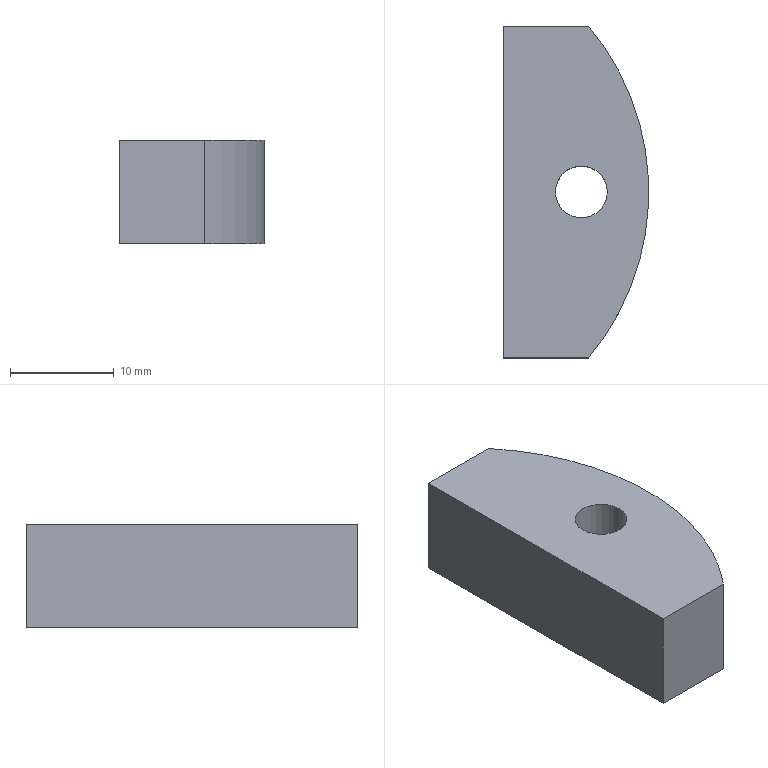Component | NX | CURVED_CLAMP_BLOCK | 1 solid | 7 faces | box 14 x 32 x 10 mm | volume 3698 mm3 | plane 5 | cylinder 2 | commonest cylinder face diameters 50 x1 5 x1
STEP:
#1=CARTESIAN_POINT('',(0.,0.,0.));
#2=DIRECTION('',(0.,0.,1.));
#3=DIRECTION('',(1.,0.,0.));
#4=AXIS2_PLACEMENT_3D('',#1,#2,#3);
#5=CARTESIAN_POINT('',(33.,15.25,-21.5));
#6=VERTEX_POINT('',#5);
#7=CARTESIAN_POINT('',(33.,-16.75,-21.5));
#8=VERTEX_POINT('',#7);
#9=CARTESIAN_POINT('',(33.,15.25,-21.5));
#10=DIRECTION('',(0.,-1.,0.));
#11=VECTOR('',#10,1.);
#12=LINE('',#9,#11);
#13=CARTESIAN_POINT('',(33.,15.25,-11.5));
#14=DIRECTION('',(1.,0.,0.));
#15=DIRECTION('',(-0.,1.,0.));
#16=AXIS2_PLACEMENT_3D('',#13,#14,#15);
#17=PLANE('',#16);
#18=CARTESIAN_POINT('',(0.,-10.));
#19=DIRECTION('',(-1.,0.));
#20=VECTOR('',#19,1.);
#21=LINE('',#18,#20);
#22=(GEOMETRIC_REPRESENTATION_CONTEXT(2)PARAMETRIC_REPRESENTATION_CONTEXT()REPRESENTATION_CONTEXT('',''));
#23=DEFINITIONAL_REPRESENTATION('',(#21),#22);
#24=PCURVE('',#17,#23);
#25=CARTESIAN_POINT('',(22.,-0.75,-21.5));
#26=DIRECTION('',(0.,0.,1.));
#27=DIRECTION('',(1.,0.,0.));
#28=AXIS2_PLACEMENT_3D('',#25,#26,#27);
#29=PLANE('',#28);
#30=CARTESIAN_POINT('',(11.,16.));
#31=DIRECTION('',(0.,-1.));
#32=VECTOR('',#31,1.);
#33=LINE('',#30,#32);
#34=(GEOMETRIC_REPRESENTATION_CONTEXT(2)PARAMETRIC_REPRESENTATION_CONTEXT()REPRESENTATION_CONTEXT('',''));
#35=DEFINITIONAL_REPRESENTATION('',(#33),#34);
#36=PCURVE('',#29,#35);
#37=SURFACE_CURVE('',#12,(#24,#36),.PCURVE_S1.);
#38=EDGE_CURVE('',#6,#8,#37,.T.);
#39=ORIENTED_EDGE('',*,*,#38,.T.);
#40=CARTESIAN_POINT('',(33.,-16.75,-11.5));
#41=VERTEX_POINT('',#40);
#42=CARTESIAN_POINT('',(33.,-16.75,-11.5));
#43=DIRECTION('',(0.,0.,-1.));
#44=VECTOR('',#43,1.);
#45=LINE('',#42,#44);
#46=CARTESIAN_POINT('',(-32.,0.));
#47=DIRECTION('',(0.,-1.));
#48=VECTOR('',#47,1.);
#49=LINE('',#46,#48);
#50=(GEOMETRIC_REPRESENTATION_CONTEXT(2)PARAMETRIC_REPRESENTATION_CONTEXT()REPRESENTATION_CONTEXT('',''));
#51=DEFINITIONAL_REPRESENTATION('',(#49),#50);
#52=PCURVE('',#17,#51);
#53=CARTESIAN_POINT('',(33.,-16.75,-11.5));
#54=DIRECTION('',(0.,1.,0.));
#55=DIRECTION('',(0.,0.,1.));
#56=AXIS2_PLACEMENT_3D('',#53,#54,#55);
#57=PLANE('',#56);
#58=CARTESIAN_POINT('',(0.,0.));
#59=DIRECTION('',(-1.,0.));
#60=VECTOR('',#59,1.);
#61=LINE('',#58,#60);
#62=(GEOMETRIC_REPRESENTATION_CONTEXT(2)PARAMETRIC_REPRESENTATION_CONTEXT()REPRESENTATION_CONTEXT('',''));
#63=DEFINITIONAL_REPRESENTATION('',(#61),#62);
#64=PCURVE('',#57,#63);
#65=SURFACE_CURVE('',#45,(#52,#64),.PCURVE_S1.);
#66=EDGE_CURVE('',#41,#8,#65,.T.);
#67=ORIENTED_EDGE('',*,*,#66,.F.);
#68=CARTESIAN_POINT('',(33.,15.25,-11.5));
#69=VERTEX_POINT('',#68);
#70=CARTESIAN_POINT('',(33.,15.25,-11.5));
#71=DIRECTION('',(0.,-1.,0.));
#72=VECTOR('',#71,1.);
#73=LINE('',#70,#72);
#74=CARTESIAN_POINT('',(0.,0.));
#75=DIRECTION('',(-1.,0.));
#76=VECTOR('',#75,1.);
#77=LINE('',#74,#76);
#78=(GEOMETRIC_REPRESENTATION_CONTEXT(2)PARAMETRIC_REPRESENTATION_CONTEXT()REPRESENTATION_CONTEXT('',''));
#79=DEFINITIONAL_REPRESENTATION('',(#77),#78);
#80=PCURVE('',#17,#79);
#81=CARTESIAN_POINT('',(22.,-0.75,-11.5));
#82=DIRECTION('',(0.,0.,1.));
#83=DIRECTION('',(1.,0.,0.));
#84=AXIS2_PLACEMENT_3D('',#81,#82,#83);
#85=PLANE('',#84);
#86=CARTESIAN_POINT('',(11.,16.));
#87=DIRECTION('',(0.,-1.));
#88=VECTOR('',#87,1.);
#89=LINE('',#86,#88);
#90=(GEOMETRIC_REPRESENTATION_CONTEXT(2)PARAMETRIC_REPRESENTATION_CONTEXT()REPRESENTATION_CONTEXT('',''));
#91=DEFINITIONAL_REPRESENTATION('',(#89),#90);
#92=PCURVE('',#85,#91);
#93=SURFACE_CURVE('',#73,(#80,#92),.PCURVE_S1.);
#94=EDGE_CURVE('',#69,#41,#93,.T.);
#95=ORIENTED_EDGE('',*,*,#94,.F.);
#96=CARTESIAN_POINT('',(33.,15.25,-11.5));
#97=DIRECTION('',(0.,0.,-1.));
#98=VECTOR('',#97,1.);
#99=LINE('',#96,#98);
#100=CARTESIAN_POINT('',(0.,0.));
#101=DIRECTION('',(0.,-1.));
#102=VECTOR('',#101,1.);
#103=LINE('',#100,#102);
#104=(GEOMETRIC_REPRESENTATION_CONTEXT(2)PARAMETRIC_REPRESENTATION_CONTEXT()REPRESENTATION_CONTEXT('',''));
#105=DEFINITIONAL_REPRESENTATION('',(#103),#104);
#106=PCURVE('',#17,#105);
#107=CARTESIAN_POINT('',(41.209,15.25,-11.5));
#108=DIRECTION('',(0.,-1.,0.));
#109=DIRECTION('',(0.,0.,-1.));
#110=AXIS2_PLACEMENT_3D('',#107,#108,#109);
#111=PLANE('',#110);
#112=CARTESIAN_POINT('',(0.,-8.209));
#113=DIRECTION('',(1.,0.));
#114=VECTOR('',#113,1.);
#115=LINE('',#112,#114);
#116=(GEOMETRIC_REPRESENTATION_CONTEXT(2)PARAMETRIC_REPRESENTATION_CONTEXT()REPRESENTATION_CONTEXT('',''));
#117=DEFINITIONAL_REPRESENTATION('',(#115),#116);
#118=PCURVE('',#111,#117);
#119=SURFACE_CURVE('',#99,(#106,#118),.PCURVE_S1.);
#120=EDGE_CURVE('',#69,#6,#119,.T.);
#121=ORIENTED_EDGE('',*,*,#120,.T.);
#122=EDGE_LOOP('',(#39,#67,#95,#121));
#123=FACE_BOUND('',#122,.T.);
#124=ADVANCED_FACE('',(#123),#17,.F.);
#125=CARTESIAN_POINT('',(41.209,-16.75,-21.5));
#126=VERTEX_POINT('',#125);
#127=CARTESIAN_POINT('',(33.,-16.75,-21.5));
#128=DIRECTION('',(1.,0.,0.));
#129=VECTOR('',#128,1.);
#130=LINE('',#127,#129);
#131=CARTESIAN_POINT('',(-10.,0.));
#132=DIRECTION('',(0.,1.));
#133=VECTOR('',#132,1.);
#134=LINE('',#131,#133);
#135=(GEOMETRIC_REPRESENTATION_CONTEXT(2)PARAMETRIC_REPRESENTATION_CONTEXT()REPRESENTATION_CONTEXT('',''));
#136=DEFINITIONAL_REPRESENTATION('',(#134),#135);
#137=PCURVE('',#57,#136);
#138=CARTESIAN_POINT('',(11.,-16.));
#139=DIRECTION('',(1.,0.));
#140=VECTOR('',#139,1.);
#141=LINE('',#138,#140);
#142=(GEOMETRIC_REPRESENTATION_CONTEXT(2)PARAMETRIC_REPRESENTATION_CONTEXT()REPRESENTATION_CONTEXT('',''));
#143=DEFINITIONAL_REPRESENTATION('',(#141),#142);
#144=PCURVE('',#29,#143);
#145=SURFACE_CURVE('',#130,(#137,#144),.PCURVE_S1.);
#146=EDGE_CURVE('',#8,#126,#145,.T.);
#147=ORIENTED_EDGE('',*,*,#146,.T.);
#148=CARTESIAN_POINT('',(41.209,-16.75,-11.5));
#149=VERTEX_POINT('',#148);
#150=CARTESIAN_POINT('',(41.209,-16.75,-11.5));
#151=DIRECTION('',(0.,0.,-1.));
#152=VECTOR('',#151,1.);
#153=LINE('',#150,#152);
#154=CARTESIAN_POINT('',(0.,8.209));
#155=DIRECTION('',(-1.,0.));
#156=VECTOR('',#155,1.);
#157=LINE('',#154,#156);
#158=(GEOMETRIC_REPRESENTATION_CONTEXT(2)PARAMETRIC_REPRESENTATION_CONTEXT()REPRESENTATION_CONTEXT('',''));
#159=DEFINITIONAL_REPRESENTATION('',(#157),#158);
#160=PCURVE('',#57,#159);
#161=CARTESIAN_POINT('',(22.,-0.75,-11.5));
#162=DIRECTION('',(0.,0.,-1.));
#163=DIRECTION('',(-1.,0.,0.));
#164=AXIS2_PLACEMENT_3D('',#161,#162,#163);
#165=CYLINDRICAL_SURFACE('',#164,25.);
#166=CARTESIAN_POINT('',(3.836,0.));
#167=DIRECTION('',(0.,1.));
#168=VECTOR('',#167,1.);
#169=LINE('',#166,#168);
#170=(GEOMETRIC_REPRESENTATION_CONTEXT(2)PARAMETRIC_REPRESENTATION_CONTEXT()REPRESENTATION_CONTEXT('',''));
#171=DEFINITIONAL_REPRESENTATION('',(#169),#170);
#172=PCURVE('',#165,#171);
#173=SURFACE_CURVE('',#153,(#160,#172),.PCURVE_S1.);
#174=EDGE_CURVE('',#149,#126,#173,.T.);
#175=ORIENTED_EDGE('',*,*,#174,.F.);
#176=CARTESIAN_POINT('',(33.,-16.75,-11.5));
#177=DIRECTION('',(1.,0.,0.));
#178=VECTOR('',#177,1.);
#179=LINE('',#176,#178);
#180=CARTESIAN_POINT('',(0.,0.));
#181=DIRECTION('',(0.,1.));
#182=VECTOR('',#181,1.);
#183=LINE('',#180,#182);
#184=(GEOMETRIC_REPRESENTATION_CONTEXT(2)PARAMETRIC_REPRESENTATION_CONTEXT()REPRESENTATION_CONTEXT('',''));
#185=DEFINITIONAL_REPRESENTATION('',(#183),#184);
#186=PCURVE('',#57,#185);
#187=CARTESIAN_POINT('',(11.,-16.));
#188=DIRECTION('',(1.,0.));
#189=VECTOR('',#188,1.);
#190=LINE('',#187,#189);
#191=(GEOMETRIC_REPRESENTATION_CONTEXT(2)PARAMETRIC_REPRESENTATION_CONTEXT()REPRESENTATION_CONTEXT('',''));
#192=DEFINITIONAL_REPRESENTATION('',(#190),#191);
#193=PCURVE('',#85,#192);
#194=SURFACE_CURVE('',#179,(#186,#193),.PCURVE_S1.);
#195=EDGE_CURVE('',#41,#149,#194,.T.);
#196=ORIENTED_EDGE('',*,*,#195,.F.);
#197=ORIENTED_EDGE('',*,*,#66,.T.);
#198=EDGE_LOOP('',(#147,#175,#196,#197));
#199=FACE_BOUND('',#198,.T.);
#200=ADVANCED_FACE('',(#199),#57,.F.);
#201=CARTESIAN_POINT('',(41.209,15.25,-21.5));
#202=VERTEX_POINT('',#201);
#203=CARTESIAN_POINT('',(22.,-0.75,-21.5));
#204=DIRECTION('',(0.,0.,1.));
#205=DIRECTION('',(1.,0.,0.));
#206=AXIS2_PLACEMENT_3D('',#203,#204,#205);
#207=CIRCLE('',#206,25.);
#208=CARTESIAN_POINT('',(9.425,10.));
#209=DIRECTION('',(-1.,0.));
#210=VECTOR('',#209,1.);
#211=LINE('',#208,#210);
#212=(GEOMETRIC_REPRESENTATION_CONTEXT(2)PARAMETRIC_REPRESENTATION_CONTEXT()REPRESENTATION_CONTEXT('',''));
#213=DEFINITIONAL_REPRESENTATION('',(#211),#212);
#214=PCURVE('',#165,#213);
#215=CARTESIAN_POINT('',(0.,0.));
#216=DIRECTION('',(1.,0.));
#217=AXIS2_PLACEMENT_2D('',#215,#216);
#218=CIRCLE('',#217,25.);
#219=(GEOMETRIC_REPRESENTATION_CONTEXT(2)PARAMETRIC_REPRESENTATION_CONTEXT()REPRESENTATION_CONTEXT('',''));
#220=DEFINITIONAL_REPRESENTATION('',(#218),#219);
#221=PCURVE('',#29,#220);
#222=SURFACE_CURVE('',#207,(#214,#221),.PCURVE_S1.);
#223=EDGE_CURVE('',#126,#202,#222,.T.);
#224=ORIENTED_EDGE('',*,*,#223,.T.);
#225=CARTESIAN_POINT('',(41.209,15.25,-11.5));
#226=VERTEX_POINT('',#225);
#227=CARTESIAN_POINT('',(41.209,15.25,-11.5));
#228=DIRECTION('',(0.,0.,-1.));
#229=VECTOR('',#228,1.);
#230=LINE('',#227,#229);
#231=CARTESIAN_POINT('',(2.447,0.));
#232=DIRECTION('',(0.,1.));
#233=VECTOR('',#232,1.);
#234=LINE('',#231,#233);
#235=(GEOMETRIC_REPRESENTATION_CONTEXT(2)PARAMETRIC_REPRESENTATION_CONTEXT()REPRESENTATION_CONTEXT('',''));
#236=DEFINITIONAL_REPRESENTATION('',(#234),#235);
#237=PCURVE('',#165,#236);
#238=CARTESIAN_POINT('',(0.,0.));
#239=DIRECTION('',(1.,0.));
#240=VECTOR('',#239,1.);
#241=LINE('',#238,#240);
#242=(GEOMETRIC_REPRESENTATION_CONTEXT(2)PARAMETRIC_REPRESENTATION_CONTEXT()REPRESENTATION_CONTEXT('',''));
#243=DEFINITIONAL_REPRESENTATION('',(#241),#242);
#244=PCURVE('',#111,#243);
#245=SURFACE_CURVE('',#230,(#237,#244),.PCURVE_S1.);
#246=EDGE_CURVE('',#226,#202,#245,.T.);
#247=ORIENTED_EDGE('',*,*,#246,.F.);
#248=CARTESIAN_POINT('',(22.,-0.75,-11.5));
#249=DIRECTION('',(0.,0.,1.));
#250=DIRECTION('',(1.,0.,0.));
#251=AXIS2_PLACEMENT_3D('',#248,#249,#250);
#252=CIRCLE('',#251,25.);
#253=CARTESIAN_POINT('',(9.425,0.));
#254=DIRECTION('',(-1.,0.));
#255=VECTOR('',#254,1.);
#256=LINE('',#253,#255);
#257=(GEOMETRIC_REPRESENTATION_CONTEXT(2)PARAMETRIC_REPRESENTATION_CONTEXT()REPRESENTATION_CONTEXT('',''));
#258=DEFINITIONAL_REPRESENTATION('',(#256),#257);
#259=PCURVE('',#165,#258);
#260=CARTESIAN_POINT('',(0.,0.));
#261=DIRECTION('',(1.,0.));
#262=AXIS2_PLACEMENT_2D('',#260,#261);
#263=CIRCLE('',#262,25.);
#264=(GEOMETRIC_REPRESENTATION_CONTEXT(2)PARAMETRIC_REPRESENTATION_CONTEXT()REPRESENTATION_CONTEXT('',''));
#265=DEFINITIONAL_REPRESENTATION('',(#263),#264);
#266=PCURVE('',#85,#265);
#267=SURFACE_CURVE('',#252,(#259,#266),.PCURVE_S1.);
#268=EDGE_CURVE('',#149,#226,#267,.T.);
#269=ORIENTED_EDGE('',*,*,#268,.F.);
#270=ORIENTED_EDGE('',*,*,#174,.T.);
#271=EDGE_LOOP('',(#224,#247,#269,#270));
#272=FACE_BOUND('',#271,.T.);
#273=ADVANCED_FACE('',(#272),#165,.T.);
#274=CARTESIAN_POINT('',(41.209,15.25,-21.5));
#275=DIRECTION('',(-1.,0.,0.));
#276=VECTOR('',#275,1.);
#277=LINE('',#274,#276);
#278=CARTESIAN_POINT('',(10.,0.));
#279=DIRECTION('',(0.,-1.));
#280=VECTOR('',#279,1.);
#281=LINE('',#278,#280);
#282=(GEOMETRIC_REPRESENTATION_CONTEXT(2)PARAMETRIC_REPRESENTATION_CONTEXT()REPRESENTATION_CONTEXT('',''));
#283=DEFINITIONAL_REPRESENTATION('',(#281),#282);
#284=PCURVE('',#111,#283);
#285=CARTESIAN_POINT('',(19.209,16.));
#286=DIRECTION('',(-1.,0.));
#287=VECTOR('',#286,1.);
#288=LINE('',#285,#287);
#289=(GEOMETRIC_REPRESENTATION_CONTEXT(2)PARAMETRIC_REPRESENTATION_CONTEXT()REPRESENTATION_CONTEXT('',''));
#290=DEFINITIONAL_REPRESENTATION('',(#288),#289);
#291=PCURVE('',#29,#290);
#292=SURFACE_CURVE('',#277,(#284,#291),.PCURVE_S1.);
#293=EDGE_CURVE('',#202,#6,#292,.T.);
#294=ORIENTED_EDGE('',*,*,#293,.T.);
#295=ORIENTED_EDGE('',*,*,#120,.F.);
#296=CARTESIAN_POINT('',(41.209,15.25,-11.5));
#297=DIRECTION('',(-1.,0.,0.));
#298=VECTOR('',#297,1.);
#299=LINE('',#296,#298);
#300=CARTESIAN_POINT('',(0.,0.));
#301=DIRECTION('',(0.,-1.));
#302=VECTOR('',#301,1.);
#303=LINE('',#300,#302);
#304=(GEOMETRIC_REPRESENTATION_CONTEXT(2)PARAMETRIC_REPRESENTATION_CONTEXT()REPRESENTATION_CONTEXT('',''));
#305=DEFINITIONAL_REPRESENTATION('',(#303),#304);
#306=PCURVE('',#111,#305);
#307=CARTESIAN_POINT('',(19.209,16.));
#308=DIRECTION('',(-1.,0.));
#309=VECTOR('',#308,1.);
#310=LINE('',#307,#309);
#311=(GEOMETRIC_REPRESENTATION_CONTEXT(2)PARAMETRIC_REPRESENTATION_CONTEXT()REPRESENTATION_CONTEXT('',''));
#312=DEFINITIONAL_REPRESENTATION('',(#310),#311);
#313=PCURVE('',#85,#312);
#314=SURFACE_CURVE('',#299,(#306,#313),.PCURVE_S1.);
#315=EDGE_CURVE('',#226,#69,#314,.T.);
#316=ORIENTED_EDGE('',*,*,#315,.F.);
#317=ORIENTED_EDGE('',*,*,#246,.T.);
#318=EDGE_LOOP('',(#294,#295,#316,#317));
#319=FACE_BOUND('',#318,.T.);
#320=ADVANCED_FACE('',(#319),#111,.F.);
#321=CARTESIAN_POINT('',(43.,-0.75,-11.5));
#322=VERTEX_POINT('',#321);
#323=CARTESIAN_POINT('',(40.5,-0.75,-11.5));
#324=DIRECTION('',(0.,0.,1.));
#325=DIRECTION('',(1.,0.,0.));
#326=AXIS2_PLACEMENT_3D('',#323,#324,#325);
#327=CIRCLE('',#326,2.5);
#328=CARTESIAN_POINT('',(40.5,-0.75,-11.5));
#329=DIRECTION('',(0.,0.,-1.));
#330=DIRECTION('',(-1.,0.,0.));
#331=AXIS2_PLACEMENT_3D('',#328,#329,#330);
#332=CYLINDRICAL_SURFACE('',#331,2.5);
#333=CARTESIAN_POINT('',(9.425,0.));
#334=DIRECTION('',(-1.,0.));
#335=VECTOR('',#334,1.);
#336=LINE('',#333,#335);
#337=(GEOMETRIC_REPRESENTATION_CONTEXT(2)PARAMETRIC_REPRESENTATION_CONTEXT()REPRESENTATION_CONTEXT('',''));
#338=DEFINITIONAL_REPRESENTATION('',(#336),#337);
#339=PCURVE('',#332,#338);
#340=CARTESIAN_POINT('',(18.5,0.));
#341=DIRECTION('',(1.,0.));
#342=AXIS2_PLACEMENT_2D('',#340,#341);
#343=CIRCLE('',#342,2.5);
#344=(GEOMETRIC_REPRESENTATION_CONTEXT(2)PARAMETRIC_REPRESENTATION_CONTEXT()REPRESENTATION_CONTEXT('',''));
#345=DEFINITIONAL_REPRESENTATION('',(#343),#344);
#346=PCURVE('',#85,#345);
#347=SURFACE_CURVE('',#327,(#339,#346),.PCURVE_S1.);
#348=EDGE_CURVE('',#322,#322,#347,.T.);
#349=ORIENTED_EDGE('',*,*,#348,.F.);
#350=CARTESIAN_POINT('',(43.,-0.75,-21.5));
#351=VERTEX_POINT('',#350);
#352=CARTESIAN_POINT('',(43.,-0.75,-11.5));
#353=CARTESIAN_POINT('',(43.,-0.75,-21.5));
#354=B_SPLINE_CURVE_WITH_KNOTS('',1,(#352,#353),.UNSPECIFIED.,.F.,.F.,(2,2),(0.,10.),.PIECEWISE_BEZIER_KNOTS.);
#355=CARTESIAN_POINT('',(9.425,0.));
#356=DIRECTION('',(0.,1.));
#357=VECTOR('',#356,1.);
#358=LINE('',#355,#357);
#359=(GEOMETRIC_REPRESENTATION_CONTEXT(2)PARAMETRIC_REPRESENTATION_CONTEXT()REPRESENTATION_CONTEXT('',''));
#360=DEFINITIONAL_REPRESENTATION('',(#358),#359);
#361=PCURVE('',#332,#360);
#362=CARTESIAN_POINT('',(3.142,0.));
#363=DIRECTION('',(0.,1.));
#364=VECTOR('',#363,1.);
#365=LINE('',#362,#364);
#366=(GEOMETRIC_REPRESENTATION_CONTEXT(2)PARAMETRIC_REPRESENTATION_CONTEXT()REPRESENTATION_CONTEXT('',''));
#367=DEFINITIONAL_REPRESENTATION('',(#365),#366);
#368=PCURVE('',#332,#367);
#369=SEAM_CURVE('',#354,(#361,#368),.PCURVE_S1.);
#370=EDGE_CURVE('',#322,#351,#369,.T.);
#371=ORIENTED_EDGE('',*,*,#370,.T.);
#372=CARTESIAN_POINT('',(40.5,-0.75,-21.5));
#373=DIRECTION('',(0.,0.,1.));
#374=DIRECTION('',(1.,0.,0.));
#375=AXIS2_PLACEMENT_3D('',#372,#373,#374);
#376=CIRCLE('',#375,2.5);
#377=CARTESIAN_POINT('',(9.425,10.));
#378=DIRECTION('',(-1.,0.));
#379=VECTOR('',#378,1.);
#380=LINE('',#377,#379);
#381=(GEOMETRIC_REPRESENTATION_CONTEXT(2)PARAMETRIC_REPRESENTATION_CONTEXT()REPRESENTATION_CONTEXT('',''));
#382=DEFINITIONAL_REPRESENTATION('',(#380),#381);
#383=PCURVE('',#332,#382);
#384=CARTESIAN_POINT('',(18.5,0.));
#385=DIRECTION('',(1.,0.));
#386=AXIS2_PLACEMENT_2D('',#384,#385);
#387=CIRCLE('',#386,2.5);
#388=(GEOMETRIC_REPRESENTATION_CONTEXT(2)PARAMETRIC_REPRESENTATION_CONTEXT()REPRESENTATION_CONTEXT('',''));
#389=DEFINITIONAL_REPRESENTATION('',(#387),#388);
#390=PCURVE('',#29,#389);
#391=SURFACE_CURVE('',#376,(#383,#390),.PCURVE_S1.);
#392=EDGE_CURVE('',#351,#351,#391,.T.);
#393=ORIENTED_EDGE('',*,*,#392,.T.);
#394=ORIENTED_EDGE('',*,*,#370,.F.);
#395=EDGE_LOOP('',(#349,#371,#393,#394));
#396=FACE_BOUND('',#395,.F.);
#397=ADVANCED_FACE('',(#396),#332,.F.);
#398=ORIENTED_EDGE('',*,*,#94,.T.);
#399=ORIENTED_EDGE('',*,*,#195,.T.);
#400=ORIENTED_EDGE('',*,*,#268,.T.);
#401=ORIENTED_EDGE('',*,*,#315,.T.);
#402=EDGE_LOOP('',(#398,#399,#400,#401));
#403=FACE_BOUND('',#402,.T.);
#404=ORIENTED_EDGE('',*,*,#348,.F.);
#405=EDGE_LOOP('',(#404));
#406=FACE_BOUND('',#405,.T.);
#407=ADVANCED_FACE('',(#403,#406),#85,.T.);
#408=ORIENTED_EDGE('',*,*,#38,.F.);
#409=ORIENTED_EDGE('',*,*,#293,.F.);
#410=ORIENTED_EDGE('',*,*,#223,.F.);
#411=ORIENTED_EDGE('',*,*,#146,.F.);
#412=EDGE_LOOP('',(#408,#409,#410,#411));
#413=FACE_BOUND('',#412,.T.);
#414=ORIENTED_EDGE('',*,*,#392,.T.);
#415=EDGE_LOOP('',(#414));
#416=FACE_BOUND('',#415,.T.);
#417=ADVANCED_FACE('',(#413,#416),#29,.F.);
#418=CLOSED_SHELL('',(#124,#200,#273,#320,#397,#407,#417));
#419=MANIFOLD_SOLID_BREP('',#418);
#420=(LENGTH_UNIT()NAMED_UNIT(*)SI_UNIT(.MILLI.,.METRE.));
#421=UNCERTAINTY_MEASURE_WITH_UNIT(LENGTH_MEASURE(0.000002),#420,'','');
#422=(NAMED_UNIT(*)PLANE_ANGLE_UNIT()SI_UNIT($,.RADIAN.));
#423=(NAMED_UNIT(*)SI_UNIT($,.STERADIAN.)SOLID_ANGLE_UNIT());
#424=(GEOMETRIC_REPRESENTATION_CONTEXT(3)GLOBAL_UNCERTAINTY_ASSIGNED_CONTEXT((#421))GLOBAL_UNIT_ASSIGNED_CONTEXT((#420,#422,#423))REPRESENTATION_CONTEXT('',''));
#425=ADVANCED_BREP_SHAPE_REPRESENTATION('',(#4,#419),#424);